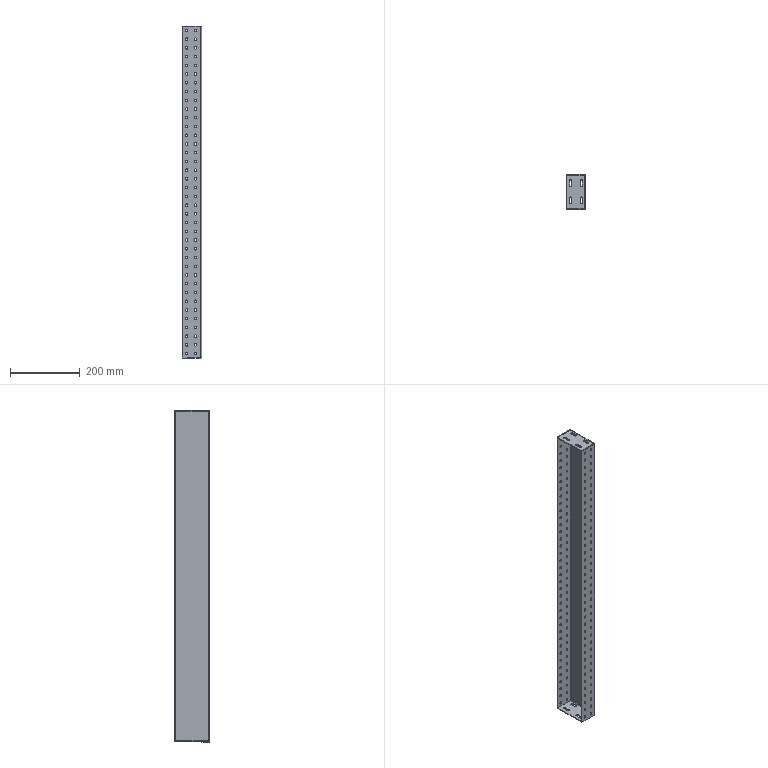Component | SolidWorks | MountingColumnMiddle-1 | 1 solid | 382 faces | volume 392331 mm3 | cylinder 336 | plane 38 | spline 8 | commonest cylinder face diameters 7 x328 8 x4 4 x4